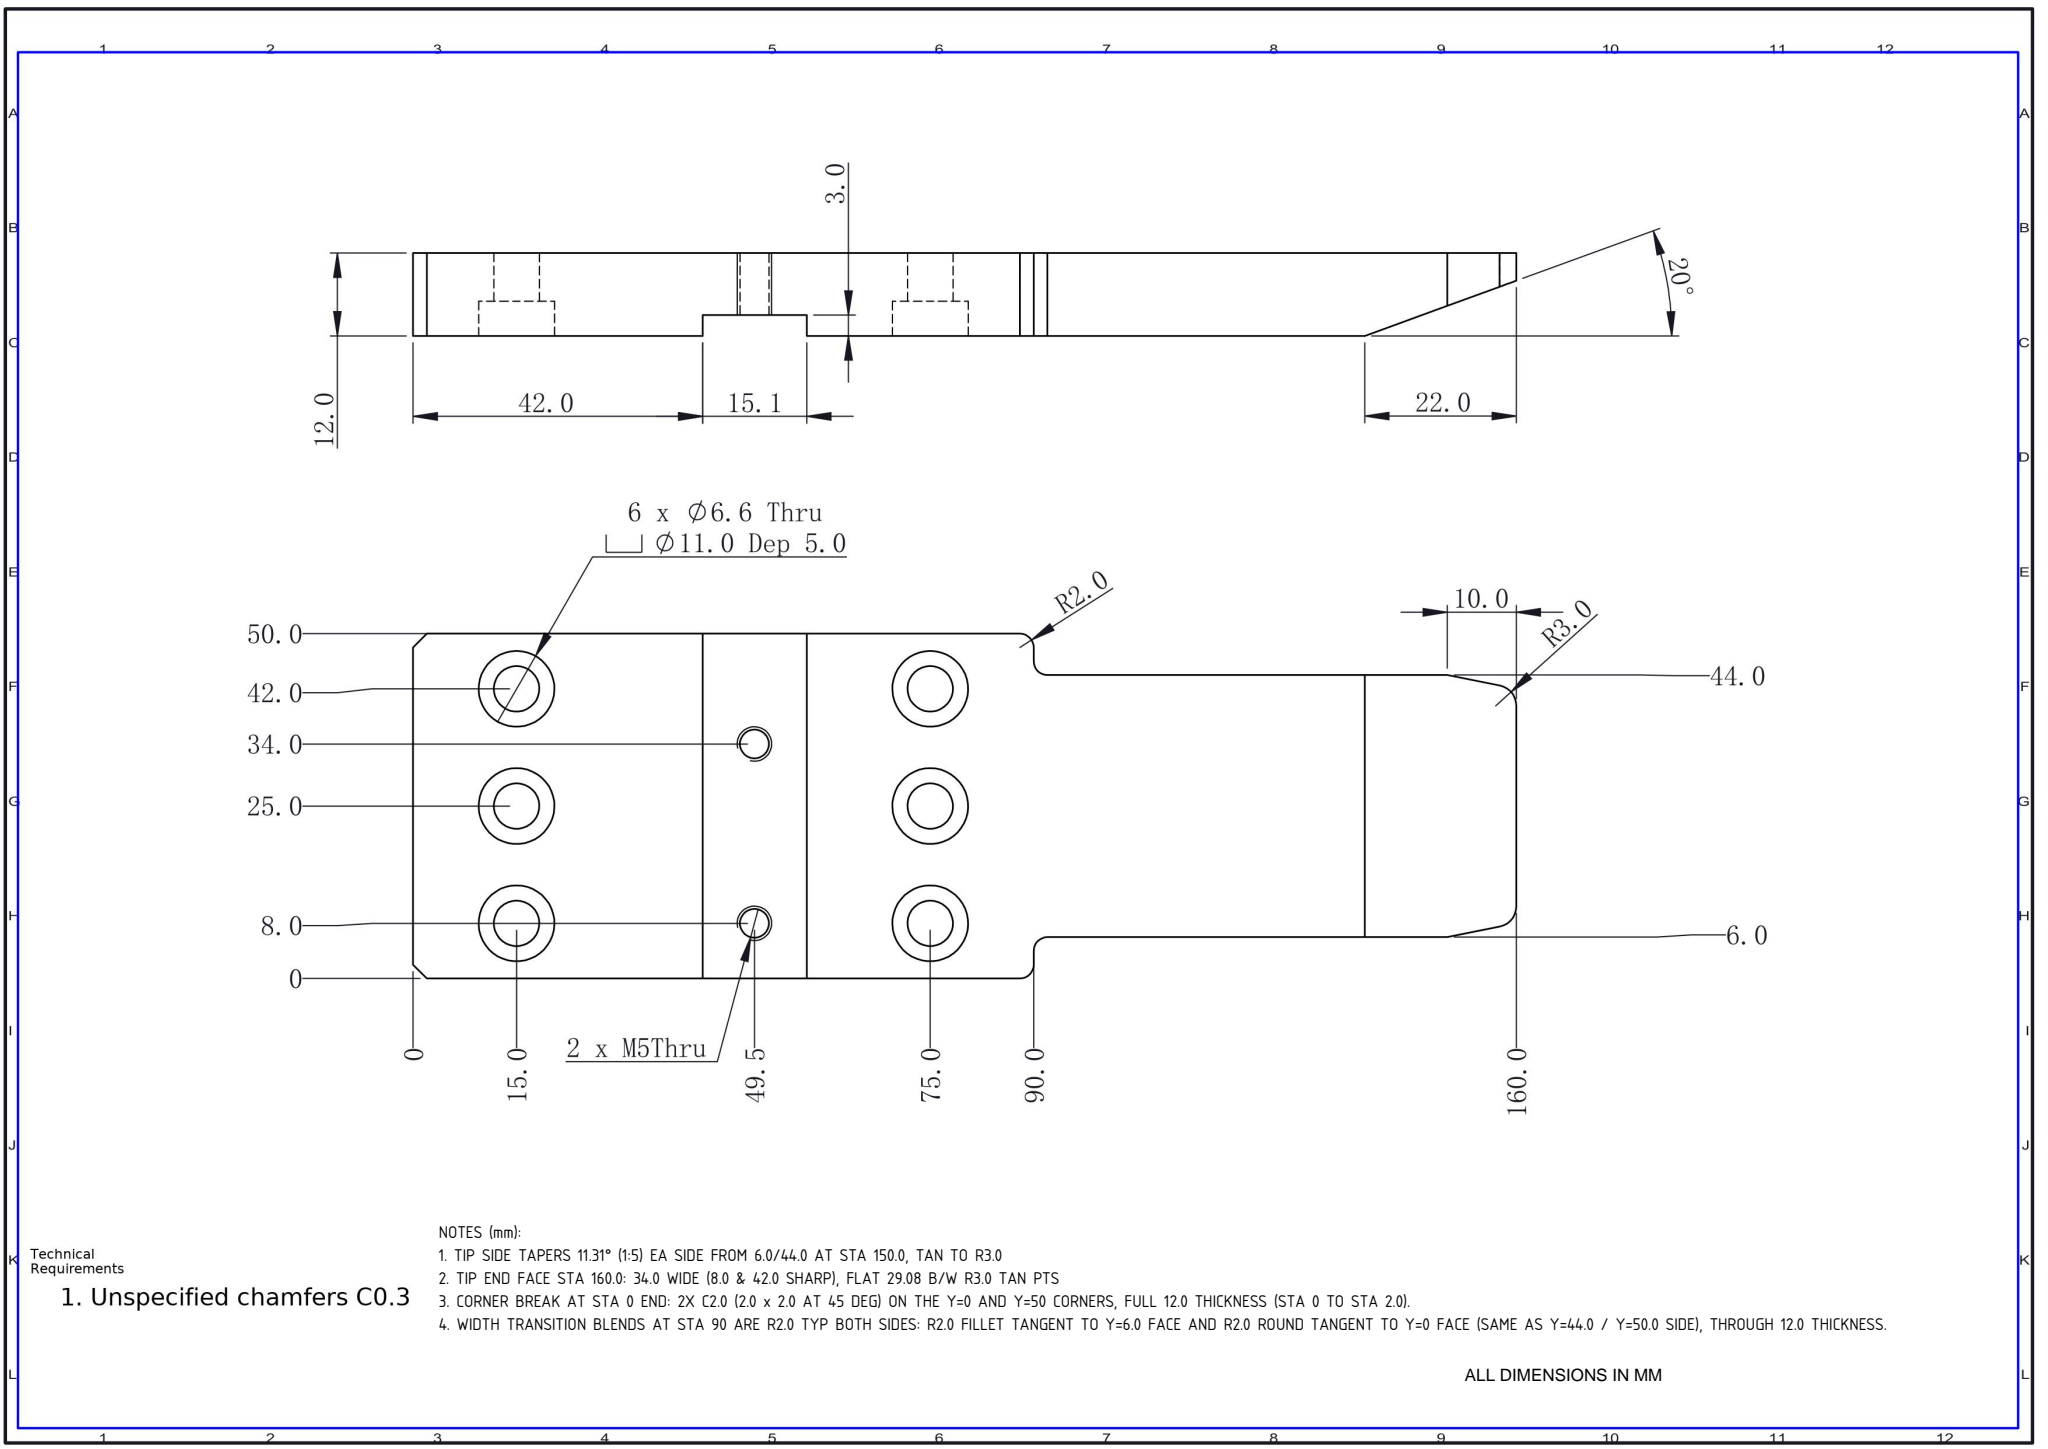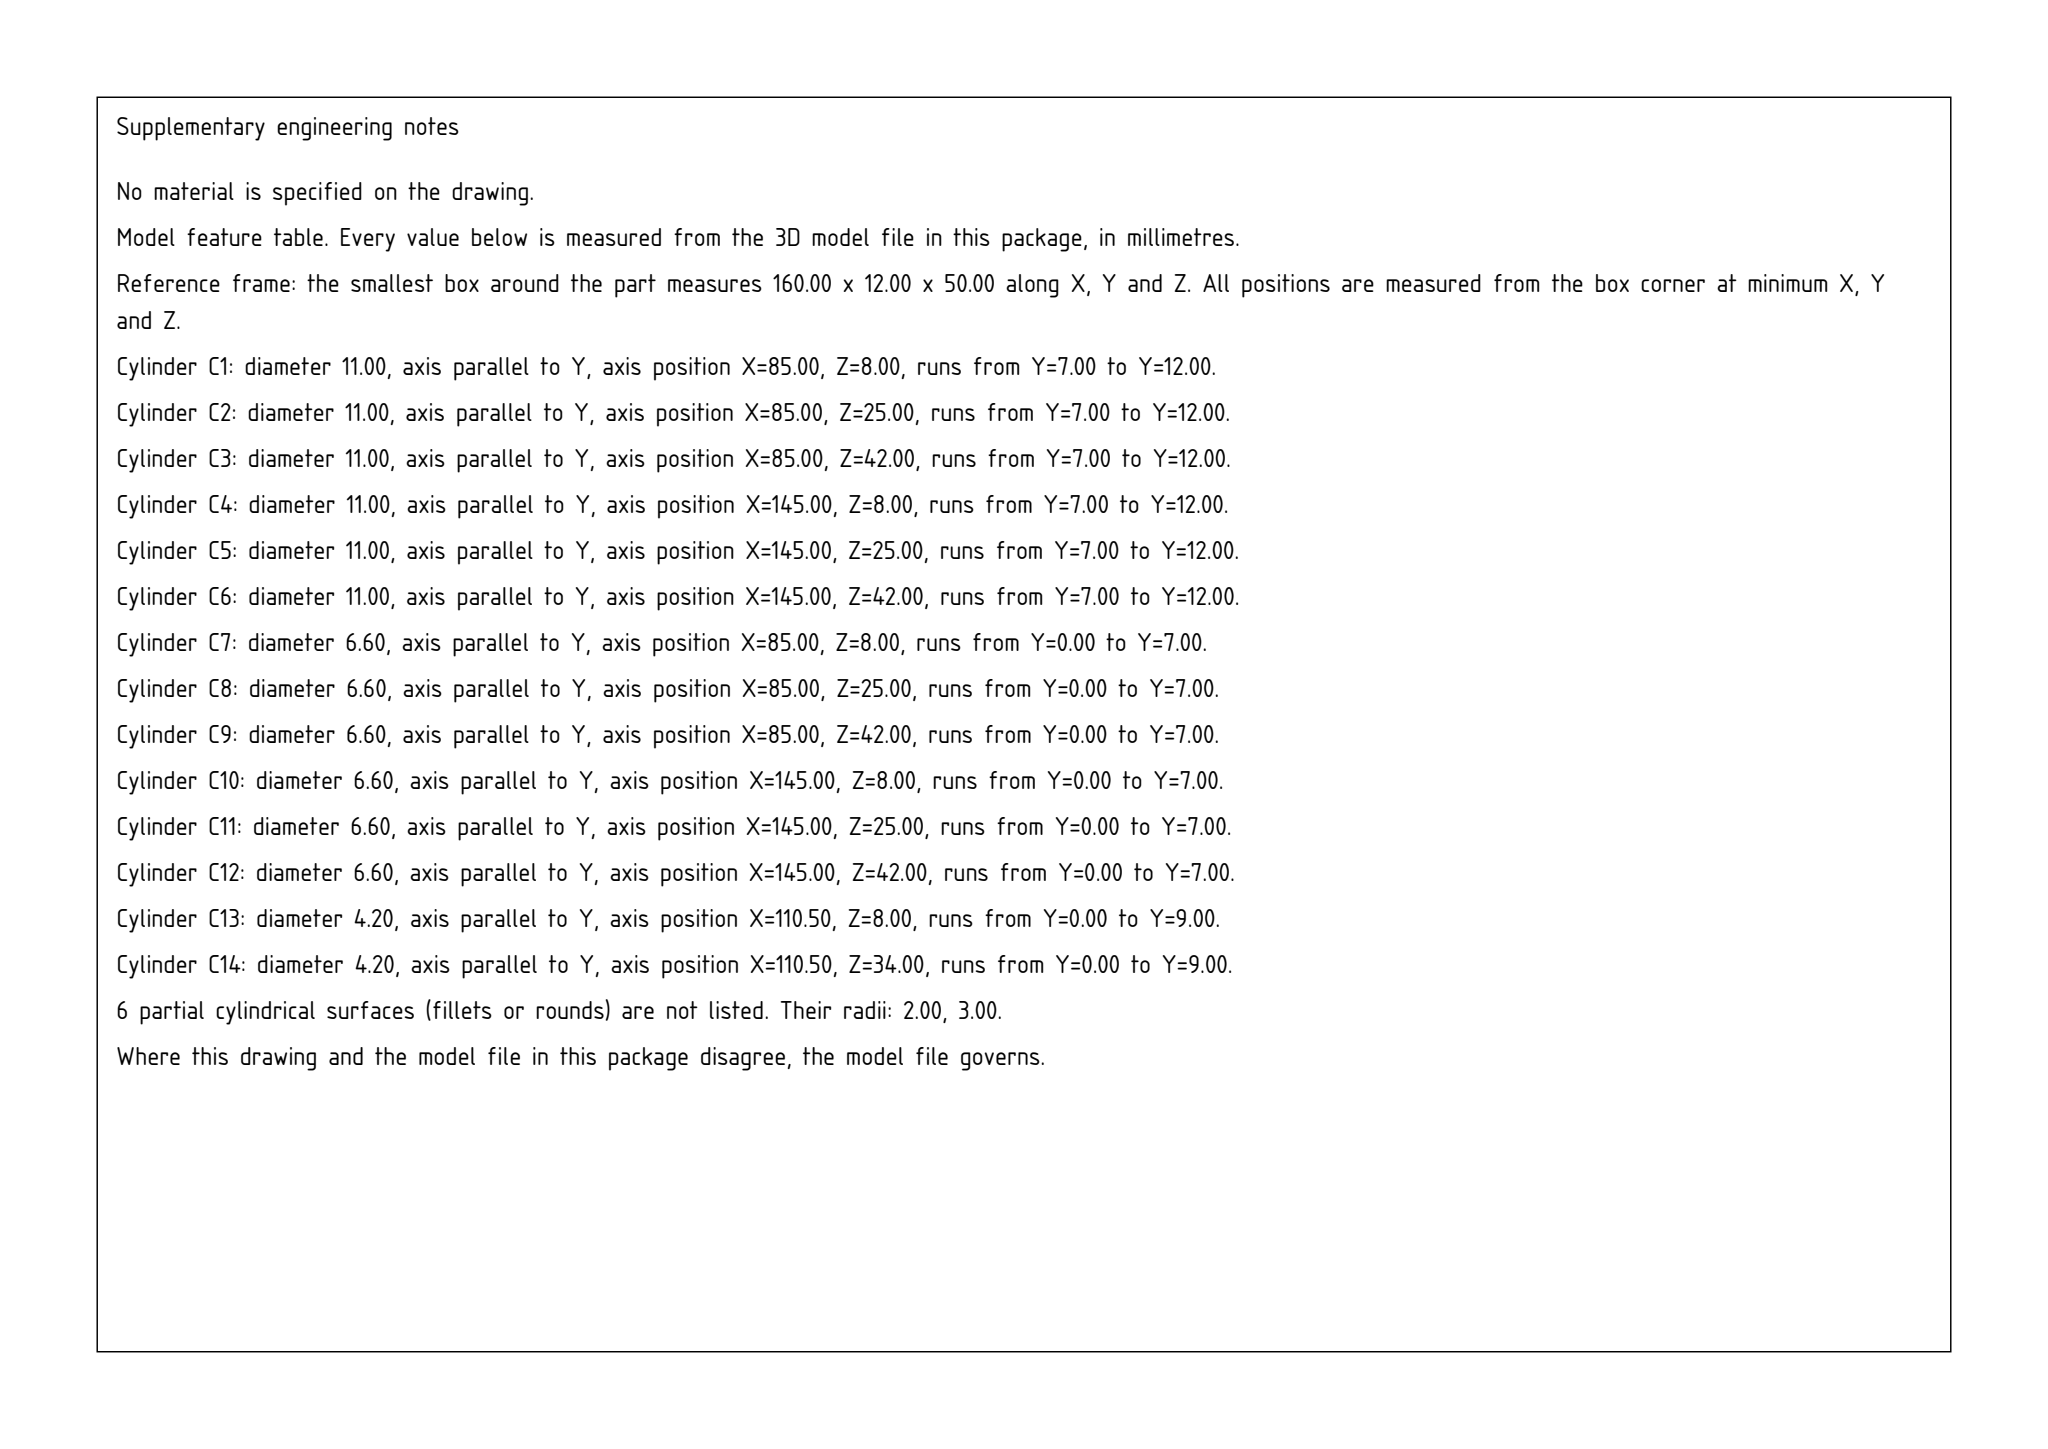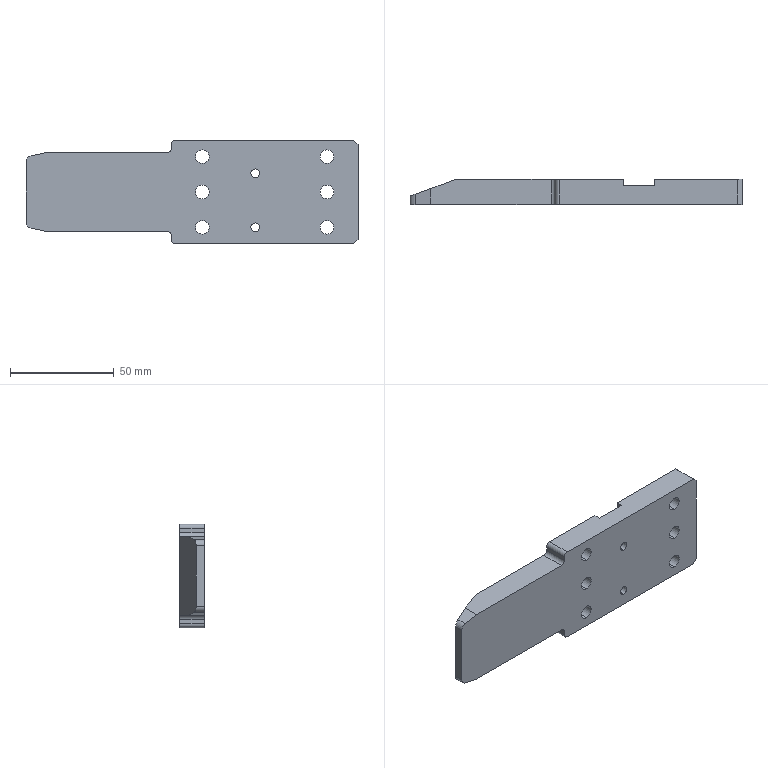Part | SolidWorks | mm | 1 solid | 59 faces | box 160 x 12 x 50 mm | volume 75614 mm3 | cylinder 34 | plane 25 | commonest cylinder face diameters 11 x12 6.6 x12 4.2 x4 4 x4 6 x2
Drawing notes:
TIP SIDE TAPERS 11.31° (1:5) EA SIDE FROM 6.0/44.0 AT STA 150.0, TAN TO R3.0 | from the solid: Edges z=6.0/44.0 end at x=10 (=STA 150.0, the 10.0 dim); tangent to R3.0 arcs centered (x=3, z=10.46/39.54) gives slope 0.2 => 11.31 deg each side
TIP END FACE STA 160.0: 34.0 WIDE (8.0 & 42.0 SHARP), FLAT 29.08 B/W R3.0 TAN PTS | from the solid: R3.0 blend cyls dia6 axis Y at x=3 (=STA 157.0), z=10.46 & 39.54; end plane x=0 (=STA 160.0); tangent lines extend to sharp corners z=8.0 & 42.0 -> 34.0 wide; flat face 29.08 between tangent pts
CORNER BREAK AT STA 0 END: 2X C2.0 (2.0 x 2.0 AT 45 DEG) ON THE Y=0 AND Y=50 CORNERS, FULL 12.0 THICKNESS (STA 0 TO STA 2.0). | from the solid: inclined_planes: angle_to_xyz_axes [45.0,90.0,45.0], bbox_from [158.0,0.0,0.0] and [158.0,0.0,48.0], size [2.0,12.0,2.0] (STEP x=158-160 = STA 0-2.0, z=0 and z=48-50)
WIDTH TRANSITION BLENDS AT STA 90 ARE R2.0 TYP BOTH SIDES: R2.0 FILLET TANGENT TO Y=6.0 FACE AND R2.0 ROUND TANGENT TO Y=0 FACE (SAME AS Y=44.0 / Y=50.0 SIDE), THROUGH 12.0 THICKNESS. | from the solid: cylinders: concave arc dia 4.0 axis y at [68.0,null,4.0] and convex arc dia 4.0 axis y at [72.0,null,2.0], y from 0.0 to 12.0, 90 deg (mirrors concave [68.0,null,46.0] / convex [72.0,null,48.0])
build123d program:
from build123d import *

# Parameters (mm, degrees)
SKETCH1_W                                       = 160
SKETCH1_H                                       = 50
BOSS_EXTRUDE1_DEPTH                             = 6
M6_HEX_SOCKET_HEAD_CAP_SCREW_CBORE1_D           = 6.6
M6_HEX_SOCKET_HEAD_CAP_SCREW_CBORE1_CBORE_D     = 11
M6_HEX_SOCKET_HEAD_CAP_SCREW_CBORE1_CBORE_DEPTH = 5
SKETCH9_W                                       = 70
SKETCH9_H                                       = 6
CUT_EXTRUDE2_DEPTH                              = 85.67
FILLET1_R                                       = 2
CHAMFER1_SIZE                                   = 2
CHAMFER1_SIZE2                                  = 10
FILLET2_R                                       = 3
CHAMFER2_SIZE                                   = 2
CUT_EXTRUDE3_DEPTH                              = 92.499
SKETCH12_W                                      = 15.1
SKETCH12_H                                      = 50
CUT_EXTRUDE4_DEPTH                              = 3
M5_TAPPED_HOLE1_D                               = 4.2


with BuildPart() as part:
    # Sketch1 → Boss-Extrude1 (new, symmetric)
    with BuildSketch(Plane(origin=(0, 0, 0), x_dir=(1, 0, 0), z_dir=(0, 1, 0))):
        Rectangle(SKETCH1_W, SKETCH1_H)
    extrude(amount=BOSS_EXTRUDE1_DEPTH, both=True)

    # M6 Hex Socket Head Cap Screw CBORE1 (through all)
    with Locations(Plane(origin=(0, 6, 0), x_dir=(1, 0, 0), z_dir=(0, 1, 0))):
        with Locations((5, 17), (65, 17), (65, -17), (5, -17), (5, 0), (65, 0)):
            CounterBoreHole(M6_HEX_SOCKET_HEAD_CAP_SCREW_CBORE1_D / 2, M6_HEX_SOCKET_HEAD_CAP_SCREW_CBORE1_CBORE_D / 2, M6_HEX_SOCKET_HEAD_CAP_SCREW_CBORE1_CBORE_DEPTH)

    # Sketch9 → Cut-Extrude2 (cut, through all)
    with BuildSketch(Plane(origin=(0, 6, 0), x_dir=(1, 0, 0), z_dir=(0, 1, 0))):
        with Locations((-45, -22)):
            Rectangle(SKETCH9_W, SKETCH9_H)
        with Locations((-45, 22)):
            Rectangle(SKETCH9_W, SKETCH9_H)
    extrude(amount=-CUT_EXTRUDE2_DEPTH, mode=Mode.SUBTRACT)

    # Fillet1
    fillet1_edges = [part.edges().sort_by_distance(p)[0] for p in [
        (-10, 0, 19),
        (-10, 0, 25),
        (-10, 0, -25),
        (-10, 0, -19),
    ]]
    fillet(fillet1_edges, radius=FILLET1_R)

    # Chamfer1
    chamfer1_edges = [part.edges().sort_by_distance(p)[0] for p in [
        (-80, 0, 19),
        (-80, 0, -19),
    ]]
    chamfer1_side = [part.faces().sort_by_distance(p)[0] for p in [
        (-80, 0, 0),
    ]]
    chamfer(chamfer1_edges, length=CHAMFER1_SIZE, length2=CHAMFER1_SIZE2, reference=chamfer1_side[0])

    # Fillet2
    fillet2_edges = [part.edges().sort_by_distance(p)[0] for p in [
        (-80, 0, -17),
        (-80, 0, 17),
    ]]
    fillet(fillet2_edges, radius=FILLET2_R)

    # Chamfer2
    chamfer2_edges = [part.edges().sort_by_distance(p)[0] for p in [
        (80, 0, 25),
        (80, 0, -25),
    ]]
    chamfer(chamfer2_edges, length=CHAMFER2_SIZE)

    # Sketch10 → Cut-Extrude3 (cut, through all)
    with BuildSketch(Plane.XY.offset(19)):
        Polygon((-80, -2), (-58.02, 6), (-80, 6), align=None)
    extrude(amount=-CUT_EXTRUDE3_DEPTH, mode=Mode.SUBTRACT)

    # Sketch12 → Cut-Extrude4 (cut)
    with BuildSketch(Plane(origin=(0, 6, 0), x_dir=(1, 0, 0), z_dir=(0, 1, 0))):
        with Locations((30.45, 0)):
            Rectangle(SKETCH12_W, SKETCH12_H)
    extrude(amount=-CUT_EXTRUDE4_DEPTH, mode=Mode.SUBTRACT)

    # M5 Tapped Hole1 (through all)
    with Locations(Plane(origin=(0, 3, 0), x_dir=(1, 0, 0), z_dir=(0, 1, 0))):
        with Locations((30.5, -9), (30.5, 17)):
            Hole(M5_TAPPED_HOLE1_D / 2)


solid = part.part